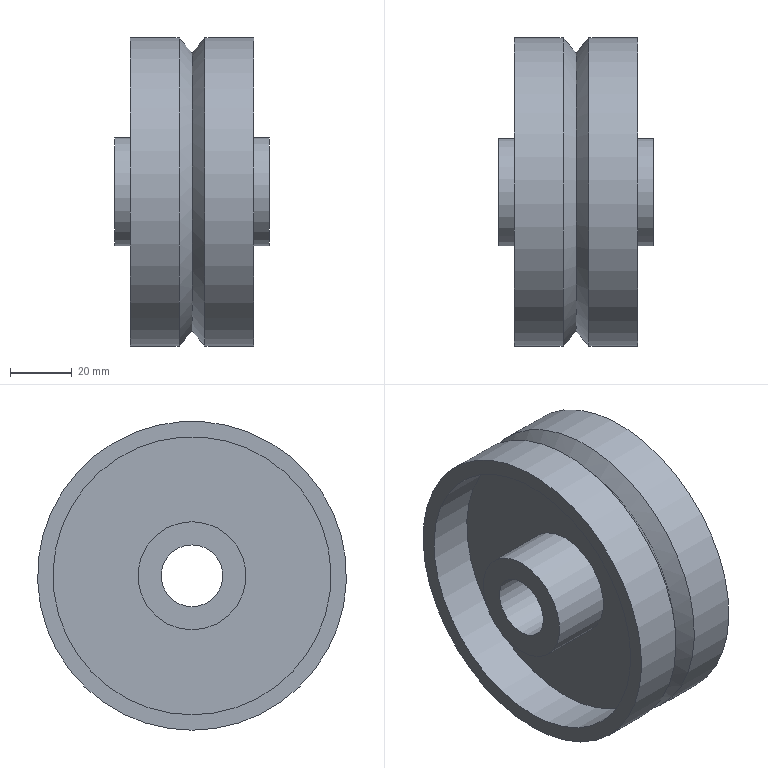Component | NX | RODA_100 | 1 solid | 15 faces | box 50 x 100 x 100 mm | volume 139713 mm3 | cylinder 7 | plane 6 | cone 2 | commonest cylinder face diameters 100 x2 90 x2 35 x2 20 x1
STEP:
#1=CARTESIAN_POINT('',(0.,0.,0.));
#2=DIRECTION('',(0.,0.,1.));
#3=DIRECTION('',(1.,0.,0.));
#4=AXIS2_PLACEMENT_3D('',#1,#2,#3);
#5=CARTESIAN_POINT('',(20.199,0.,-60.));
#6=VERTEX_POINT('',#5);
#7=CARTESIAN_POINT('',(20.199,0.,-10.));
#8=DIRECTION('',(-1.,0.,0.));
#9=DIRECTION('',(0.,0.,-1.));
#10=AXIS2_PLACEMENT_3D('',#7,#8,#9);
#11=CIRCLE('',#10,50.);
#12=CARTESIAN_POINT('',(140.199,0.,-10.));
#13=DIRECTION('',(-1.,0.,0.));
#14=DIRECTION('',(0.,0.,-1.));
#15=AXIS2_PLACEMENT_3D('',#12,#13,#14);
#16=CYLINDRICAL_SURFACE('',#15,50.);
#17=CARTESIAN_POINT('',(0.,120.));
#18=DIRECTION('',(1.,0.));
#19=VECTOR('',#18,1.);
#20=LINE('',#17,#19);
#21=(GEOMETRIC_REPRESENTATION_CONTEXT(2)PARAMETRIC_REPRESENTATION_CONTEXT()REPRESENTATION_CONTEXT('',''));
#22=DEFINITIONAL_REPRESENTATION('',(#20),#21);
#23=PCURVE('',#16,#22);
#24=CARTESIAN_POINT('',(20.199,-50.,-10.));
#25=DIRECTION('',(1.,0.,0.));
#26=DIRECTION('',(0.,0.,1.));
#27=AXIS2_PLACEMENT_3D('',#24,#25,#26);
#28=PLANE('',#27);
#29=CARTESIAN_POINT('',(-50.,-50.));
#30=CARTESIAN_POINT('',(-50.,36.603));
#31=CARTESIAN_POINT('',(25.,-6.699));
#32=CARTESIAN_POINT('',(100.,-50.));
#33=CARTESIAN_POINT('',(25.,-93.301));
#34=CARTESIAN_POINT('',(-50.,-136.603));
#35=CARTESIAN_POINT('',(-50.,-50.));
#36=(BOUNDED_CURVE()B_SPLINE_CURVE(2,(#29,#30,#31,#32,#33,#34,#35),.UNSPECIFIED.,.T.,.F.)B_SPLINE_CURVE_WITH_KNOTS((1,2,2,2,2,1),(-2.094,0.,2.094,4.189,6.283,8.378),.UNSPECIFIED.)CURVE()GEOMETRIC_REPRESENTATION_ITEM()RATIONAL_B_SPLINE_CURVE((1.,0.5,1.,0.5,1.,0.5,1.))REPRESENTATION_ITEM(''));
#37=(GEOMETRIC_REPRESENTATION_CONTEXT(2)PARAMETRIC_REPRESENTATION_CONTEXT()REPRESENTATION_CONTEXT('',''));
#38=DEFINITIONAL_REPRESENTATION('',(#36),#37);
#39=PCURVE('',#28,#38);
#40=SURFACE_CURVE('',#11,(#23,#39),.PCURVE_S1.);
#41=EDGE_CURVE('',#6,#6,#40,.T.);
#42=ORIENTED_EDGE('',*,*,#41,.T.);
#43=CARTESIAN_POINT('',(4.394,0.,-60.));
#44=VERTEX_POINT('',#43);
#45=CARTESIAN_POINT('',(20.199,0.,-60.));
#46=CARTESIAN_POINT('',(4.394,0.,-60.));
#47=B_SPLINE_CURVE_WITH_KNOTS('',1,(#45,#46),.UNSPECIFIED.,.F.,.F.,(2,2),(120.,135.805),.PIECEWISE_BEZIER_KNOTS.);
#48=CARTESIAN_POINT('',(6.283,0.));
#49=DIRECTION('',(0.,1.));
#50=VECTOR('',#49,1.);
#51=LINE('',#48,#50);
#52=(GEOMETRIC_REPRESENTATION_CONTEXT(2)PARAMETRIC_REPRESENTATION_CONTEXT()REPRESENTATION_CONTEXT('',''));
#53=DEFINITIONAL_REPRESENTATION('',(#51),#52);
#54=PCURVE('',#16,#53);
#55=CARTESIAN_POINT('',(0.,0.));
#56=DIRECTION('',(0.,1.));
#57=VECTOR('',#56,1.);
#58=LINE('',#55,#57);
#59=(GEOMETRIC_REPRESENTATION_CONTEXT(2)PARAMETRIC_REPRESENTATION_CONTEXT()REPRESENTATION_CONTEXT('',''));
#60=DEFINITIONAL_REPRESENTATION('',(#58),#59);
#61=PCURVE('',#16,#60);
#62=SEAM_CURVE('',#47,(#54,#61),.PCURVE_S1.);
#63=EDGE_CURVE('',#6,#44,#62,.T.);
#64=ORIENTED_EDGE('',*,*,#63,.T.);
#65=CARTESIAN_POINT('',(4.394,0.,-10.));
#66=DIRECTION('',(-1.,0.,0.));
#67=DIRECTION('',(0.,0.,-1.));
#68=AXIS2_PLACEMENT_3D('',#65,#66,#67);
#69=CIRCLE('',#68,50.);
#70=CARTESIAN_POINT('',(0.,135.805));
#71=DIRECTION('',(1.,0.));
#72=VECTOR('',#71,1.);
#73=LINE('',#70,#72);
#74=(GEOMETRIC_REPRESENTATION_CONTEXT(2)PARAMETRIC_REPRESENTATION_CONTEXT()REPRESENTATION_CONTEXT('',''));
#75=DEFINITIONAL_REPRESENTATION('',(#73),#74);
#76=PCURVE('',#16,#75);
#77=CARTESIAN_POINT('',(0.1986,0.,-10.));
#78=DIRECTION('',(1.,0.,0.));
#79=DIRECTION('',(0.,0.,1.));
#80=AXIS2_PLACEMENT_3D('',#77,#78,#79);
#81=CONICAL_SURFACE('',#80,45.,0.8727);
#82=CARTESIAN_POINT('',(9.425,4.195));
#83=DIRECTION('',(-1.,0.));
#84=VECTOR('',#83,1.);
#85=LINE('',#82,#84);
#86=(GEOMETRIC_REPRESENTATION_CONTEXT(2)PARAMETRIC_REPRESENTATION_CONTEXT()REPRESENTATION_CONTEXT('',''));
#87=DEFINITIONAL_REPRESENTATION('',(#85),#86);
#88=PCURVE('',#81,#87);
#89=SURFACE_CURVE('',#69,(#76,#88),.PCURVE_S1.);
#90=EDGE_CURVE('',#44,#44,#89,.T.);
#91=ORIENTED_EDGE('',*,*,#90,.F.);
#92=ORIENTED_EDGE('',*,*,#63,.F.);
#93=EDGE_LOOP('',(#42,#64,#91,#92));
#94=FACE_BOUND('',#93,.T.);
#95=ADVANCED_FACE('',(#94),#16,.T.);
#96=CARTESIAN_POINT('',(20.199,0.,-55.));
#97=VERTEX_POINT('',#96);
#98=CARTESIAN_POINT('',(20.199,0.,-10.));
#99=DIRECTION('',(-1.,0.,0.));
#100=DIRECTION('',(0.,0.,-1.));
#101=AXIS2_PLACEMENT_3D('',#98,#99,#100);
#102=CIRCLE('',#101,45.);
#103=CARTESIAN_POINT('',(-45.,-50.));
#104=CARTESIAN_POINT('',(-45.,27.942));
#105=CARTESIAN_POINT('',(22.5,-11.029));
#106=CARTESIAN_POINT('',(90.,-50.));
#107=CARTESIAN_POINT('',(22.5,-88.971));
#108=CARTESIAN_POINT('',(-45.,-127.942));
#109=CARTESIAN_POINT('',(-45.,-50.));
#110=(BOUNDED_CURVE()B_SPLINE_CURVE(2,(#103,#104,#105,#106,#107,#108,#109),.UNSPECIFIED.,.T.,.F.)B_SPLINE_CURVE_WITH_KNOTS((1,2,2,2,2,1),(-2.094,0.,2.094,4.189,6.283,8.378),.UNSPECIFIED.)CURVE()GEOMETRIC_REPRESENTATION_ITEM()RATIONAL_B_SPLINE_CURVE((1.,0.5,1.,0.5,1.,0.5,1.))REPRESENTATION_ITEM(''));
#111=(GEOMETRIC_REPRESENTATION_CONTEXT(2)PARAMETRIC_REPRESENTATION_CONTEXT()REPRESENTATION_CONTEXT('',''));
#112=DEFINITIONAL_REPRESENTATION('',(#110),#111);
#113=PCURVE('',#28,#112);
#114=CARTESIAN_POINT('',(140.199,0.,-10.));
#115=DIRECTION('',(-1.,0.,0.));
#116=DIRECTION('',(0.,0.,-1.));
#117=AXIS2_PLACEMENT_3D('',#114,#115,#116);
#118=CYLINDRICAL_SURFACE('',#117,45.);
#119=CARTESIAN_POINT('',(0.,120.));
#120=DIRECTION('',(1.,0.));
#121=VECTOR('',#120,1.);
#122=LINE('',#119,#121);
#123=(GEOMETRIC_REPRESENTATION_CONTEXT(2)PARAMETRIC_REPRESENTATION_CONTEXT()REPRESENTATION_CONTEXT('',''));
#124=DEFINITIONAL_REPRESENTATION('',(#122),#123);
#125=PCURVE('',#118,#124);
#126=SURFACE_CURVE('',#102,(#113,#125),.PCURVE_S1.);
#127=EDGE_CURVE('',#97,#97,#126,.T.);
#128=ORIENTED_EDGE('',*,*,#127,.T.);
#129=EDGE_LOOP('',(#128));
#130=FACE_BOUND('',#129,.T.);
#131=ORIENTED_EDGE('',*,*,#41,.F.);
#132=EDGE_LOOP('',(#131));
#133=FACE_BOUND('',#132,.T.);
#134=ADVANCED_FACE('',(#130,#133),#28,.T.);
#135=CARTESIAN_POINT('',(5.199,0.,-55.));
#136=VERTEX_POINT('',#135);
#137=CARTESIAN_POINT('',(5.199,0.,-10.));
#138=DIRECTION('',(-1.,0.,0.));
#139=DIRECTION('',(0.,0.,-1.));
#140=AXIS2_PLACEMENT_3D('',#137,#138,#139);
#141=CIRCLE('',#140,45.);
#142=CARTESIAN_POINT('',(0.,135.));
#143=DIRECTION('',(1.,0.));
#144=VECTOR('',#143,1.);
#145=LINE('',#142,#144);
#146=(GEOMETRIC_REPRESENTATION_CONTEXT(2)PARAMETRIC_REPRESENTATION_CONTEXT()REPRESENTATION_CONTEXT('',''));
#147=DEFINITIONAL_REPRESENTATION('',(#145),#146);
#148=PCURVE('',#118,#147);
#149=CARTESIAN_POINT('',(5.199,-45.,-10.));
#150=DIRECTION('',(1.,0.,0.));
#151=DIRECTION('',(0.,0.,1.));
#152=AXIS2_PLACEMENT_3D('',#149,#150,#151);
#153=PLANE('',#152);
#154=CARTESIAN_POINT('',(-45.,-45.));
#155=CARTESIAN_POINT('',(-45.,32.942));
#156=CARTESIAN_POINT('',(22.5,-6.029));
#157=CARTESIAN_POINT('',(90.,-45.));
#158=CARTESIAN_POINT('',(22.5,-83.971));
#159=CARTESIAN_POINT('',(-45.,-122.942));
#160=CARTESIAN_POINT('',(-45.,-45.));
#161=(BOUNDED_CURVE()B_SPLINE_CURVE(2,(#154,#155,#156,#157,#158,#159,#160),.UNSPECIFIED.,.T.,.F.)B_SPLINE_CURVE_WITH_KNOTS((1,2,2,2,2,1),(-2.094,0.,2.094,4.189,6.283,8.378),.UNSPECIFIED.)CURVE()GEOMETRIC_REPRESENTATION_ITEM()RATIONAL_B_SPLINE_CURVE((1.,0.5,1.,0.5,1.,0.5,1.))REPRESENTATION_ITEM(''));
#162=(GEOMETRIC_REPRESENTATION_CONTEXT(2)PARAMETRIC_REPRESENTATION_CONTEXT()REPRESENTATION_CONTEXT('',''));
#163=DEFINITIONAL_REPRESENTATION('',(#161),#162);
#164=PCURVE('',#153,#163);
#165=SURFACE_CURVE('',#141,(#148,#164),.PCURVE_S1.);
#166=EDGE_CURVE('',#136,#136,#165,.T.);
#167=ORIENTED_EDGE('',*,*,#166,.F.);
#168=CARTESIAN_POINT('',(20.199,0.,-55.));
#169=CARTESIAN_POINT('',(5.199,0.,-55.));
#170=B_SPLINE_CURVE_WITH_KNOTS('',1,(#168,#169),.UNSPECIFIED.,.F.,.F.,(2,2),(120.,135.),.PIECEWISE_BEZIER_KNOTS.);
#171=CARTESIAN_POINT('',(0.,0.));
#172=DIRECTION('',(0.,1.));
#173=VECTOR('',#172,1.);
#174=LINE('',#171,#173);
#175=(GEOMETRIC_REPRESENTATION_CONTEXT(2)PARAMETRIC_REPRESENTATION_CONTEXT()REPRESENTATION_CONTEXT('',''));
#176=DEFINITIONAL_REPRESENTATION('',(#174),#175);
#177=PCURVE('',#118,#176);
#178=CARTESIAN_POINT('',(6.283,0.));
#179=DIRECTION('',(0.,1.));
#180=VECTOR('',#179,1.);
#181=LINE('',#178,#180);
#182=(GEOMETRIC_REPRESENTATION_CONTEXT(2)PARAMETRIC_REPRESENTATION_CONTEXT()REPRESENTATION_CONTEXT('',''));
#183=DEFINITIONAL_REPRESENTATION('',(#181),#182);
#184=PCURVE('',#118,#183);
#185=SEAM_CURVE('',#170,(#177,#184),.PCURVE_S1.);
#186=EDGE_CURVE('',#97,#136,#185,.T.);
#187=ORIENTED_EDGE('',*,*,#186,.F.);
#188=ORIENTED_EDGE('',*,*,#127,.T.);
#189=ORIENTED_EDGE('',*,*,#186,.T.);
#190=EDGE_LOOP('',(#167,#187,#188,#189));
#191=FACE_BOUND('',#190,.F.);
#192=ADVANCED_FACE('',(#191),#118,.F.);
#193=CARTESIAN_POINT('',(5.199,0.,-27.5));
#194=VERTEX_POINT('',#193);
#195=CARTESIAN_POINT('',(5.199,0.,-10.));
#196=DIRECTION('',(-1.,0.,0.));
#197=DIRECTION('',(0.,0.,-1.));
#198=AXIS2_PLACEMENT_3D('',#195,#196,#197);
#199=CIRCLE('',#198,17.5);
#200=CARTESIAN_POINT('',(-17.5,-45.));
#201=CARTESIAN_POINT('',(-17.5,-14.689));
#202=CARTESIAN_POINT('',(8.75,-29.845));
#203=CARTESIAN_POINT('',(35.,-45.));
#204=CARTESIAN_POINT('',(8.75,-60.155));
#205=CARTESIAN_POINT('',(-17.5,-75.311));
#206=CARTESIAN_POINT('',(-17.5,-45.));
#207=(BOUNDED_CURVE()B_SPLINE_CURVE(2,(#200,#201,#202,#203,#204,#205,#206),.UNSPECIFIED.,.T.,.F.)B_SPLINE_CURVE_WITH_KNOTS((1,2,2,2,2,1),(-2.094,0.,2.094,4.189,6.283,8.378),.UNSPECIFIED.)CURVE()GEOMETRIC_REPRESENTATION_ITEM()RATIONAL_B_SPLINE_CURVE((1.,0.5,1.,0.5,1.,0.5,1.))REPRESENTATION_ITEM(''));
#208=(GEOMETRIC_REPRESENTATION_CONTEXT(2)PARAMETRIC_REPRESENTATION_CONTEXT()REPRESENTATION_CONTEXT('',''));
#209=DEFINITIONAL_REPRESENTATION('',(#207),#208);
#210=PCURVE('',#153,#209);
#211=CARTESIAN_POINT('',(140.199,0.,-10.));
#212=DIRECTION('',(-1.,0.,0.));
#213=DIRECTION('',(0.,0.,-1.));
#214=AXIS2_PLACEMENT_3D('',#211,#212,#213);
#215=CYLINDRICAL_SURFACE('',#214,17.5);
#216=CARTESIAN_POINT('',(0.,135.));
#217=DIRECTION('',(1.,0.));
#218=VECTOR('',#217,1.);
#219=LINE('',#216,#218);
#220=(GEOMETRIC_REPRESENTATION_CONTEXT(2)PARAMETRIC_REPRESENTATION_CONTEXT()REPRESENTATION_CONTEXT('',''));
#221=DEFINITIONAL_REPRESENTATION('',(#219),#220);
#222=PCURVE('',#215,#221);
#223=SURFACE_CURVE('',#199,(#210,#222),.PCURVE_S1.);
#224=EDGE_CURVE('',#194,#194,#223,.T.);
#225=ORIENTED_EDGE('',*,*,#224,.T.);
#226=EDGE_LOOP('',(#225));
#227=FACE_BOUND('',#226,.T.);
#228=ORIENTED_EDGE('',*,*,#166,.F.);
#229=EDGE_LOOP('',(#228));
#230=FACE_BOUND('',#229,.T.);
#231=ADVANCED_FACE('',(#227,#230),#153,.T.);
#232=CARTESIAN_POINT('',(25.199,0.,-27.5));
#233=VERTEX_POINT('',#232);
#234=CARTESIAN_POINT('',(25.199,0.,-10.));
#235=DIRECTION('',(-1.,0.,0.));
#236=DIRECTION('',(0.,0.,-1.));
#237=AXIS2_PLACEMENT_3D('',#234,#235,#236);
#238=CIRCLE('',#237,17.5);
#239=CARTESIAN_POINT('',(0.,115.));
#240=DIRECTION('',(1.,0.));
#241=VECTOR('',#240,1.);
#242=LINE('',#239,#241);
#243=(GEOMETRIC_REPRESENTATION_CONTEXT(2)PARAMETRIC_REPRESENTATION_CONTEXT()REPRESENTATION_CONTEXT('',''));
#244=DEFINITIONAL_REPRESENTATION('',(#242),#243);
#245=PCURVE('',#215,#244);
#246=CARTESIAN_POINT('',(25.199,-17.5,-10.));
#247=DIRECTION('',(1.,0.,0.));
#248=DIRECTION('',(0.,0.,1.));
#249=AXIS2_PLACEMENT_3D('',#246,#247,#248);
#250=PLANE('',#249);
#251=CARTESIAN_POINT('',(-17.5,-17.5));
#252=CARTESIAN_POINT('',(-17.5,12.811));
#253=CARTESIAN_POINT('',(8.75,-2.345));
#254=CARTESIAN_POINT('',(35.,-17.5));
#255=CARTESIAN_POINT('',(8.75,-32.655));
#256=CARTESIAN_POINT('',(-17.5,-47.811));
#257=CARTESIAN_POINT('',(-17.5,-17.5));
#258=(BOUNDED_CURVE()B_SPLINE_CURVE(2,(#251,#252,#253,#254,#255,#256,#257),.UNSPECIFIED.,.T.,.F.)B_SPLINE_CURVE_WITH_KNOTS((1,2,2,2,2,1),(-2.094,0.,2.094,4.189,6.283,8.378),.UNSPECIFIED.)CURVE()GEOMETRIC_REPRESENTATION_ITEM()RATIONAL_B_SPLINE_CURVE((1.,0.5,1.,0.5,1.,0.5,1.))REPRESENTATION_ITEM(''));
#259=(GEOMETRIC_REPRESENTATION_CONTEXT(2)PARAMETRIC_REPRESENTATION_CONTEXT()REPRESENTATION_CONTEXT('',''));
#260=DEFINITIONAL_REPRESENTATION('',(#258),#259);
#261=PCURVE('',#250,#260);
#262=SURFACE_CURVE('',#238,(#245,#261),.PCURVE_S1.);
#263=EDGE_CURVE('',#233,#233,#262,.T.);
#264=ORIENTED_EDGE('',*,*,#263,.T.);
#265=CARTESIAN_POINT('',(25.199,0.,-27.5));
#266=CARTESIAN_POINT('',(5.199,0.,-27.5));
#267=B_SPLINE_CURVE_WITH_KNOTS('',1,(#265,#266),.UNSPECIFIED.,.F.,.F.,(2,2),(115.,135.),.PIECEWISE_BEZIER_KNOTS.);
#268=CARTESIAN_POINT('',(6.283,0.));
#269=DIRECTION('',(0.,1.));
#270=VECTOR('',#269,1.);
#271=LINE('',#268,#270);
#272=(GEOMETRIC_REPRESENTATION_CONTEXT(2)PARAMETRIC_REPRESENTATION_CONTEXT()REPRESENTATION_CONTEXT('',''));
#273=DEFINITIONAL_REPRESENTATION('',(#271),#272);
#274=PCURVE('',#215,#273);
#275=CARTESIAN_POINT('',(0.,0.));
#276=DIRECTION('',(0.,1.));
#277=VECTOR('',#276,1.);
#278=LINE('',#275,#277);
#279=(GEOMETRIC_REPRESENTATION_CONTEXT(2)PARAMETRIC_REPRESENTATION_CONTEXT()REPRESENTATION_CONTEXT('',''));
#280=DEFINITIONAL_REPRESENTATION('',(#278),#279);
#281=PCURVE('',#215,#280);
#282=SEAM_CURVE('',#267,(#274,#281),.PCURVE_S1.);
#283=EDGE_CURVE('',#233,#194,#282,.T.);
#284=ORIENTED_EDGE('',*,*,#283,.T.);
#285=ORIENTED_EDGE('',*,*,#224,.F.);
#286=ORIENTED_EDGE('',*,*,#283,.F.);
#287=EDGE_LOOP('',(#264,#284,#285,#286));
#288=FACE_BOUND('',#287,.T.);
#289=ADVANCED_FACE('',(#288),#215,.T.);
#290=CARTESIAN_POINT('',(25.199,0.,-20.));
#291=VERTEX_POINT('',#290);
#292=CARTESIAN_POINT('',(25.199,0.,-10.));
#293=DIRECTION('',(-1.,0.,0.));
#294=DIRECTION('',(0.,0.,-1.));
#295=AXIS2_PLACEMENT_3D('',#292,#293,#294);
#296=CIRCLE('',#295,10.);
#297=CARTESIAN_POINT('',(-10.,-17.5));
#298=CARTESIAN_POINT('',(-10.,-0.1795));
#299=CARTESIAN_POINT('',(5.,-8.84));
#300=CARTESIAN_POINT('',(20.,-17.5));
#301=CARTESIAN_POINT('',(5.,-26.16));
#302=CARTESIAN_POINT('',(-10.,-34.821));
#303=CARTESIAN_POINT('',(-10.,-17.5));
#304=(BOUNDED_CURVE()B_SPLINE_CURVE(2,(#297,#298,#299,#300,#301,#302,#303),.UNSPECIFIED.,.T.,.F.)B_SPLINE_CURVE_WITH_KNOTS((1,2,2,2,2,1),(-2.094,0.,2.094,4.189,6.283,8.378),.UNSPECIFIED.)CURVE()GEOMETRIC_REPRESENTATION_ITEM()RATIONAL_B_SPLINE_CURVE((1.,0.5,1.,0.5,1.,0.5,1.))REPRESENTATION_ITEM(''));
#305=(GEOMETRIC_REPRESENTATION_CONTEXT(2)PARAMETRIC_REPRESENTATION_CONTEXT()REPRESENTATION_CONTEXT('',''));
#306=DEFINITIONAL_REPRESENTATION('',(#304),#305);
#307=PCURVE('',#250,#306);
#308=CARTESIAN_POINT('',(140.199,0.,-10.));
#309=DIRECTION('',(-1.,0.,0.));
#310=DIRECTION('',(0.,0.,-1.));
#311=AXIS2_PLACEMENT_3D('',#308,#309,#310);
#312=CYLINDRICAL_SURFACE('',#311,10.);
#313=CARTESIAN_POINT('',(0.,115.));
#314=DIRECTION('',(1.,0.));
#315=VECTOR('',#314,1.);
#316=LINE('',#313,#315);
#317=(GEOMETRIC_REPRESENTATION_CONTEXT(2)PARAMETRIC_REPRESENTATION_CONTEXT()REPRESENTATION_CONTEXT('',''));
#318=DEFINITIONAL_REPRESENTATION('',(#316),#317);
#319=PCURVE('',#312,#318);
#320=SURFACE_CURVE('',#296,(#307,#319),.PCURVE_S1.);
#321=EDGE_CURVE('',#291,#291,#320,.T.);
#322=ORIENTED_EDGE('',*,*,#321,.T.);
#323=EDGE_LOOP('',(#322));
#324=FACE_BOUND('',#323,.T.);
#325=ORIENTED_EDGE('',*,*,#263,.F.);
#326=EDGE_LOOP('',(#325));
#327=FACE_BOUND('',#326,.T.);
#328=ADVANCED_FACE('',(#324,#327),#250,.T.);
#329=CARTESIAN_POINT('',(-24.801,0.,-20.));
#330=VERTEX_POINT('',#329);
#331=CARTESIAN_POINT('',(-24.801,0.,-10.));
#332=DIRECTION('',(-1.,0.,0.));
#333=DIRECTION('',(0.,0.,-1.));
#334=AXIS2_PLACEMENT_3D('',#331,#332,#333);
#335=CIRCLE('',#334,10.);
#336=CARTESIAN_POINT('',(0.,165.));
#337=DIRECTION('',(1.,0.));
#338=VECTOR('',#337,1.);
#339=LINE('',#336,#338);
#340=(GEOMETRIC_REPRESENTATION_CONTEXT(2)PARAMETRIC_REPRESENTATION_CONTEXT()REPRESENTATION_CONTEXT('',''));
#341=DEFINITIONAL_REPRESENTATION('',(#339),#340);
#342=PCURVE('',#312,#341);
#343=CARTESIAN_POINT('',(-24.801,-10.,-10.));
#344=DIRECTION('',(-1.,0.,0.));
#345=DIRECTION('',(0.,0.,-1.));
#346=AXIS2_PLACEMENT_3D('',#343,#344,#345);
#347=PLANE('',#346);
#348=CARTESIAN_POINT('',(0.,-10.));
#349=DIRECTION('',(1.,0.));
#350=AXIS2_PLACEMENT_2D('',#348,#349);
#351=CIRCLE('',#350,10.);
#352=(GEOMETRIC_REPRESENTATION_CONTEXT(2)PARAMETRIC_REPRESENTATION_CONTEXT()REPRESENTATION_CONTEXT('',''));
#353=DEFINITIONAL_REPRESENTATION('',(#351),#352);
#354=PCURVE('',#347,#353);
#355=SURFACE_CURVE('',#335,(#342,#354),.PCURVE_S1.);
#356=EDGE_CURVE('',#330,#330,#355,.T.);
#357=ORIENTED_EDGE('',*,*,#356,.F.);
#358=CARTESIAN_POINT('',(25.199,0.,-20.));
#359=CARTESIAN_POINT('',(-24.801,0.,-20.));
#360=B_SPLINE_CURVE_WITH_KNOTS('',1,(#358,#359),.UNSPECIFIED.,.F.,.F.,(2,2),(115.,165.),.PIECEWISE_BEZIER_KNOTS.);
#361=CARTESIAN_POINT('',(0.,0.));
#362=DIRECTION('',(0.,1.));
#363=VECTOR('',#362,1.);
#364=LINE('',#361,#363);
#365=(GEOMETRIC_REPRESENTATION_CONTEXT(2)PARAMETRIC_REPRESENTATION_CONTEXT()REPRESENTATION_CONTEXT('',''));
#366=DEFINITIONAL_REPRESENTATION('',(#364),#365);
#367=PCURVE('',#312,#366);
#368=CARTESIAN_POINT('',(6.283,0.));
#369=DIRECTION('',(0.,1.));
#370=VECTOR('',#369,1.);
#371=LINE('',#368,#370);
#372=(GEOMETRIC_REPRESENTATION_CONTEXT(2)PARAMETRIC_REPRESENTATION_CONTEXT()REPRESENTATION_CONTEXT('',''));
#373=DEFINITIONAL_REPRESENTATION('',(#371),#372);
#374=PCURVE('',#312,#373);
#375=SEAM_CURVE('',#360,(#367,#374),.PCURVE_S1.);
#376=EDGE_CURVE('',#291,#330,#375,.T.);
#377=ORIENTED_EDGE('',*,*,#376,.F.);
#378=ORIENTED_EDGE('',*,*,#321,.T.);
#379=ORIENTED_EDGE('',*,*,#376,.T.);
#380=EDGE_LOOP('',(#357,#377,#378,#379));
#381=FACE_BOUND('',#380,.F.);
#382=ADVANCED_FACE('',(#381),#312,.F.);
#383=CARTESIAN_POINT('',(-24.801,0.,-27.5));
#384=VERTEX_POINT('',#383);
#385=CARTESIAN_POINT('',(-24.801,0.,-10.));
#386=DIRECTION('',(-1.,0.,0.));
#387=DIRECTION('',(0.,0.,-1.));
#388=AXIS2_PLACEMENT_3D('',#385,#386,#387);
#389=CIRCLE('',#388,17.5);
#390=CARTESIAN_POINT('',(0.,-10.));
#391=DIRECTION('',(1.,0.));
#392=AXIS2_PLACEMENT_2D('',#390,#391);
#393=CIRCLE('',#392,17.5);
#394=(GEOMETRIC_REPRESENTATION_CONTEXT(2)PARAMETRIC_REPRESENTATION_CONTEXT()REPRESENTATION_CONTEXT('',''));
#395=DEFINITIONAL_REPRESENTATION('',(#393),#394);
#396=PCURVE('',#347,#395);
#397=CARTESIAN_POINT('',(140.199,0.,-10.));
#398=DIRECTION('',(-1.,0.,0.));
#399=DIRECTION('',(0.,0.,-1.));
#400=AXIS2_PLACEMENT_3D('',#397,#398,#399);
#401=CYLINDRICAL_SURFACE('',#400,17.5);
#402=CARTESIAN_POINT('',(0.,165.));
#403=DIRECTION('',(1.,0.));
#404=VECTOR('',#403,1.);
#405=LINE('',#402,#404);
#406=(GEOMETRIC_REPRESENTATION_CONTEXT(2)PARAMETRIC_REPRESENTATION_CONTEXT()REPRESENTATION_CONTEXT('',''));
#407=DEFINITIONAL_REPRESENTATION('',(#405),#406);
#408=PCURVE('',#401,#407);
#409=SURFACE_CURVE('',#389,(#396,#408),.PCURVE_S1.);
#410=EDGE_CURVE('',#384,#384,#409,.T.);
#411=ORIENTED_EDGE('',*,*,#410,.T.);
#412=EDGE_LOOP('',(#411));
#413=FACE_BOUND('',#412,.T.);
#414=ORIENTED_EDGE('',*,*,#356,.F.);
#415=EDGE_LOOP('',(#414));
#416=FACE_BOUND('',#415,.T.);
#417=ADVANCED_FACE('',(#413,#416),#347,.T.);
#418=CARTESIAN_POINT('',(-4.801,0.,-27.5));
#419=VERTEX_POINT('',#418);
#420=CARTESIAN_POINT('',(-4.801,0.,-10.));
#421=DIRECTION('',(-1.,0.,0.));
#422=DIRECTION('',(0.,0.,-1.));
#423=AXIS2_PLACEMENT_3D('',#420,#421,#422);
#424=CIRCLE('',#423,17.5);
#425=CARTESIAN_POINT('',(0.,145.));
#426=DIRECTION('',(1.,0.));
#427=VECTOR('',#426,1.);
#428=LINE('',#425,#427);
#429=(GEOMETRIC_REPRESENTATION_CONTEXT(2)PARAMETRIC_REPRESENTATION_CONTEXT()REPRESENTATION_CONTEXT('',''));
#430=DEFINITIONAL_REPRESENTATION('',(#428),#429);
#431=PCURVE('',#401,#430);
#432=CARTESIAN_POINT('',(-4.801,-17.5,-10.));
#433=DIRECTION('',(-1.,0.,0.));
#434=DIRECTION('',(0.,0.,-1.));
#435=AXIS2_PLACEMENT_3D('',#432,#433,#434);
#436=PLANE('',#435);
#437=CARTESIAN_POINT('',(0.,-17.5));
#438=DIRECTION('',(1.,0.));
#439=AXIS2_PLACEMENT_2D('',#437,#438);
#440=CIRCLE('',#439,17.5);
#441=(GEOMETRIC_REPRESENTATION_CONTEXT(2)PARAMETRIC_REPRESENTATION_CONTEXT()REPRESENTATION_CONTEXT('',''));
#442=DEFINITIONAL_REPRESENTATION('',(#440),#441);
#443=PCURVE('',#436,#442);
#444=SURFACE_CURVE('',#424,(#431,#443),.PCURVE_S1.);
#445=EDGE_CURVE('',#419,#419,#444,.T.);
#446=ORIENTED_EDGE('',*,*,#445,.T.);
#447=CARTESIAN_POINT('',(-4.801,0.,-27.5));
#448=CARTESIAN_POINT('',(-24.801,0.,-27.5));
#449=B_SPLINE_CURVE_WITH_KNOTS('',1,(#447,#448),.UNSPECIFIED.,.F.,.F.,(2,2),(145.,165.),.PIECEWISE_BEZIER_KNOTS.);
#450=CARTESIAN_POINT('',(6.283,0.));
#451=DIRECTION('',(0.,1.));
#452=VECTOR('',#451,1.);
#453=LINE('',#450,#452);
#454=(GEOMETRIC_REPRESENTATION_CONTEXT(2)PARAMETRIC_REPRESENTATION_CONTEXT()REPRESENTATION_CONTEXT('',''));
#455=DEFINITIONAL_REPRESENTATION('',(#453),#454);
#456=PCURVE('',#401,#455);
#457=CARTESIAN_POINT('',(0.,0.));
#458=DIRECTION('',(0.,1.));
#459=VECTOR('',#458,1.);
#460=LINE('',#457,#459);
#461=(GEOMETRIC_REPRESENTATION_CONTEXT(2)PARAMETRIC_REPRESENTATION_CONTEXT()REPRESENTATION_CONTEXT('',''));
#462=DEFINITIONAL_REPRESENTATION('',(#460),#461);
#463=PCURVE('',#401,#462);
#464=SEAM_CURVE('',#449,(#456,#463),.PCURVE_S1.);
#465=EDGE_CURVE('',#419,#384,#464,.T.);
#466=ORIENTED_EDGE('',*,*,#465,.T.);
#467=ORIENTED_EDGE('',*,*,#410,.F.);
#468=ORIENTED_EDGE('',*,*,#465,.F.);
#469=EDGE_LOOP('',(#446,#466,#467,#468));
#470=FACE_BOUND('',#469,.T.);
#471=ADVANCED_FACE('',(#470),#401,.T.);
#472=CARTESIAN_POINT('',(-4.801,0.,-55.));
#473=VERTEX_POINT('',#472);
#474=CARTESIAN_POINT('',(-4.801,0.,-10.));
#475=DIRECTION('',(-1.,0.,0.));
#476=DIRECTION('',(0.,0.,-1.));
#477=AXIS2_PLACEMENT_3D('',#474,#475,#476);
#478=CIRCLE('',#477,45.);
#479=CARTESIAN_POINT('',(0.,-17.5));
#480=DIRECTION('',(1.,0.));
#481=AXIS2_PLACEMENT_2D('',#479,#480);
#482=CIRCLE('',#481,45.);
#483=(GEOMETRIC_REPRESENTATION_CONTEXT(2)PARAMETRIC_REPRESENTATION_CONTEXT()REPRESENTATION_CONTEXT('',''));
#484=DEFINITIONAL_REPRESENTATION('',(#482),#483);
#485=PCURVE('',#436,#484);
#486=CARTESIAN_POINT('',(140.199,0.,-10.));
#487=DIRECTION('',(-1.,0.,0.));
#488=DIRECTION('',(0.,0.,-1.));
#489=AXIS2_PLACEMENT_3D('',#486,#487,#488);
#490=CYLINDRICAL_SURFACE('',#489,45.);
#491=CARTESIAN_POINT('',(0.,145.));
#492=DIRECTION('',(1.,0.));
#493=VECTOR('',#492,1.);
#494=LINE('',#491,#493);
#495=(GEOMETRIC_REPRESENTATION_CONTEXT(2)PARAMETRIC_REPRESENTATION_CONTEXT()REPRESENTATION_CONTEXT('',''));
#496=DEFINITIONAL_REPRESENTATION('',(#494),#495);
#497=PCURVE('',#490,#496);
#498=SURFACE_CURVE('',#478,(#485,#497),.PCURVE_S1.);
#499=EDGE_CURVE('',#473,#473,#498,.T.);
#500=ORIENTED_EDGE('',*,*,#499,.T.);
#501=EDGE_LOOP('',(#500));
#502=FACE_BOUND('',#501,.T.);
#503=ORIENTED_EDGE('',*,*,#445,.F.);
#504=EDGE_LOOP('',(#503));
#505=FACE_BOUND('',#504,.T.);
#506=ADVANCED_FACE('',(#502,#505),#436,.T.);
#507=CARTESIAN_POINT('',(-19.801,0.,-55.));
#508=VERTEX_POINT('',#507);
#509=CARTESIAN_POINT('',(-19.801,0.,-10.));
#510=DIRECTION('',(-1.,0.,0.));
#511=DIRECTION('',(0.,0.,-1.));
#512=AXIS2_PLACEMENT_3D('',#509,#510,#511);
#513=CIRCLE('',#512,45.);
#514=CARTESIAN_POINT('',(0.,160.));
#515=DIRECTION('',(1.,0.));
#516=VECTOR('',#515,1.);
#517=LINE('',#514,#516);
#518=(GEOMETRIC_REPRESENTATION_CONTEXT(2)PARAMETRIC_REPRESENTATION_CONTEXT()REPRESENTATION_CONTEXT('',''));
#519=DEFINITIONAL_REPRESENTATION('',(#517),#518);
#520=PCURVE('',#490,#519);
#521=CARTESIAN_POINT('',(-19.801,-45.,-10.));
#522=DIRECTION('',(-1.,0.,0.));
#523=DIRECTION('',(0.,0.,-1.));
#524=AXIS2_PLACEMENT_3D('',#521,#522,#523);
#525=PLANE('',#524);
#526=CARTESIAN_POINT('',(0.,-45.));
#527=DIRECTION('',(1.,0.));
#528=AXIS2_PLACEMENT_2D('',#526,#527);
#529=CIRCLE('',#528,45.);
#530=(GEOMETRIC_REPRESENTATION_CONTEXT(2)PARAMETRIC_REPRESENTATION_CONTEXT()REPRESENTATION_CONTEXT('',''));
#531=DEFINITIONAL_REPRESENTATION('',(#529),#530);
#532=PCURVE('',#525,#531);
#533=SURFACE_CURVE('',#513,(#520,#532),.PCURVE_S1.);
#534=EDGE_CURVE('',#508,#508,#533,.T.);
#535=ORIENTED_EDGE('',*,*,#534,.F.);
#536=CARTESIAN_POINT('',(-4.801,0.,-55.));
#537=CARTESIAN_POINT('',(-19.801,0.,-55.));
#538=B_SPLINE_CURVE_WITH_KNOTS('',1,(#536,#537),.UNSPECIFIED.,.F.,.F.,(2,2),(145.,160.),.PIECEWISE_BEZIER_KNOTS.);
#539=CARTESIAN_POINT('',(0.,0.));
#540=DIRECTION('',(0.,1.));
#541=VECTOR('',#540,1.);
#542=LINE('',#539,#541);
#543=(GEOMETRIC_REPRESENTATION_CONTEXT(2)PARAMETRIC_REPRESENTATION_CONTEXT()REPRESENTATION_CONTEXT('',''));
#544=DEFINITIONAL_REPRESENTATION('',(#542),#543);
#545=PCURVE('',#490,#544);
#546=CARTESIAN_POINT('',(6.283,0.));
#547=DIRECTION('',(0.,1.));
#548=VECTOR('',#547,1.);
#549=LINE('',#546,#548);
#550=(GEOMETRIC_REPRESENTATION_CONTEXT(2)PARAMETRIC_REPRESENTATION_CONTEXT()REPRESENTATION_CONTEXT('',''));
#551=DEFINITIONAL_REPRESENTATION('',(#549),#550);
#552=PCURVE('',#490,#551);
#553=SEAM_CURVE('',#538,(#545,#552),.PCURVE_S1.);
#554=EDGE_CURVE('',#473,#508,#553,.T.);
#555=ORIENTED_EDGE('',*,*,#554,.F.);
#556=ORIENTED_EDGE('',*,*,#499,.T.);
#557=ORIENTED_EDGE('',*,*,#554,.T.);
#558=EDGE_LOOP('',(#535,#555,#556,#557));
#559=FACE_BOUND('',#558,.F.);
#560=ADVANCED_FACE('',(#559),#490,.F.);
#561=CARTESIAN_POINT('',(-19.801,0.,-60.));
#562=VERTEX_POINT('',#561);
#563=CARTESIAN_POINT('',(-19.801,0.,-10.));
#564=DIRECTION('',(-1.,0.,0.));
#565=DIRECTION('',(0.,0.,-1.));
#566=AXIS2_PLACEMENT_3D('',#563,#564,#565);
#567=CIRCLE('',#566,50.);
#568=CARTESIAN_POINT('',(0.,-45.));
#569=DIRECTION('',(1.,0.));
#570=AXIS2_PLACEMENT_2D('',#568,#569);
#571=CIRCLE('',#570,50.);
#572=(GEOMETRIC_REPRESENTATION_CONTEXT(2)PARAMETRIC_REPRESENTATION_CONTEXT()REPRESENTATION_CONTEXT('',''));
#573=DEFINITIONAL_REPRESENTATION('',(#571),#572);
#574=PCURVE('',#525,#573);
#575=CARTESIAN_POINT('',(140.199,0.,-10.));
#576=DIRECTION('',(-1.,0.,0.));
#577=DIRECTION('',(0.,0.,-1.));
#578=AXIS2_PLACEMENT_3D('',#575,#576,#577);
#579=CYLINDRICAL_SURFACE('',#578,50.);
#580=CARTESIAN_POINT('',(0.,160.));
#581=DIRECTION('',(1.,0.));
#582=VECTOR('',#581,1.);
#583=LINE('',#580,#582);
#584=(GEOMETRIC_REPRESENTATION_CONTEXT(2)PARAMETRIC_REPRESENTATION_CONTEXT()REPRESENTATION_CONTEXT('',''));
#585=DEFINITIONAL_REPRESENTATION('',(#583),#584);
#586=PCURVE('',#579,#585);
#587=SURFACE_CURVE('',#567,(#574,#586),.PCURVE_S1.);
#588=EDGE_CURVE('',#562,#562,#587,.T.);
#589=ORIENTED_EDGE('',*,*,#588,.T.);
#590=EDGE_LOOP('',(#589));
#591=FACE_BOUND('',#590,.T.);
#592=ORIENTED_EDGE('',*,*,#534,.F.);
#593=EDGE_LOOP('',(#592));
#594=FACE_BOUND('',#593,.T.);
#595=ADVANCED_FACE('',(#591,#594),#525,.T.);
#596=CARTESIAN_POINT('',(-3.997,0.,-60.));
#597=VERTEX_POINT('',#596);
#598=CARTESIAN_POINT('',(-3.997,0.,-10.));
#599=DIRECTION('',(-1.,0.,0.));
#600=DIRECTION('',(0.,0.,-1.));
#601=AXIS2_PLACEMENT_3D('',#598,#599,#600);
#602=CIRCLE('',#601,50.);
#603=CARTESIAN_POINT('',(0.,144.195));
#604=DIRECTION('',(1.,0.));
#605=VECTOR('',#604,1.);
#606=LINE('',#603,#605);
#607=(GEOMETRIC_REPRESENTATION_CONTEXT(2)PARAMETRIC_REPRESENTATION_CONTEXT()REPRESENTATION_CONTEXT('',''));
#608=DEFINITIONAL_REPRESENTATION('',(#606),#607);
#609=PCURVE('',#579,#608);
#610=CARTESIAN_POINT('',(-3.997,0.,-10.));
#611=DIRECTION('',(-1.,0.,0.));
#612=DIRECTION('',(0.,0.,-1.));
#613=AXIS2_PLACEMENT_3D('',#610,#611,#612);
#614=CONICAL_SURFACE('',#613,50.,0.8727);
#615=CARTESIAN_POINT('',(0.,0.));
#616=DIRECTION('',(1.,0.));
#617=VECTOR('',#616,1.);
#618=LINE('',#615,#617);
#619=(GEOMETRIC_REPRESENTATION_CONTEXT(2)PARAMETRIC_REPRESENTATION_CONTEXT()REPRESENTATION_CONTEXT('',''));
#620=DEFINITIONAL_REPRESENTATION('',(#618),#619);
#621=PCURVE('',#614,#620);
#622=SURFACE_CURVE('',#602,(#609,#621),.PCURVE_S1.);
#623=EDGE_CURVE('',#597,#597,#622,.T.);
#624=ORIENTED_EDGE('',*,*,#623,.T.);
#625=CARTESIAN_POINT('',(-3.997,0.,-60.));
#626=CARTESIAN_POINT('',(-19.801,0.,-60.));
#627=B_SPLINE_CURVE_WITH_KNOTS('',1,(#625,#626),.UNSPECIFIED.,.F.,.F.,(2,2),(144.195,160.),.PIECEWISE_BEZIER_KNOTS.);
#628=CARTESIAN_POINT('',(6.283,0.));
#629=DIRECTION('',(0.,1.));
#630=VECTOR('',#629,1.);
#631=LINE('',#628,#630);
#632=(GEOMETRIC_REPRESENTATION_CONTEXT(2)PARAMETRIC_REPRESENTATION_CONTEXT()REPRESENTATION_CONTEXT('',''));
#633=DEFINITIONAL_REPRESENTATION('',(#631),#632);
#634=PCURVE('',#579,#633);
#635=CARTESIAN_POINT('',(0.,0.));
#636=DIRECTION('',(0.,1.));
#637=VECTOR('',#636,1.);
#638=LINE('',#635,#637);
#639=(GEOMETRIC_REPRESENTATION_CONTEXT(2)PARAMETRIC_REPRESENTATION_CONTEXT()REPRESENTATION_CONTEXT('',''));
#640=DEFINITIONAL_REPRESENTATION('',(#638),#639);
#641=PCURVE('',#579,#640);
#642=SEAM_CURVE('',#627,(#634,#641),.PCURVE_S1.);
#643=EDGE_CURVE('',#597,#562,#642,.T.);
#644=ORIENTED_EDGE('',*,*,#643,.T.);
#645=ORIENTED_EDGE('',*,*,#588,.F.);
#646=ORIENTED_EDGE('',*,*,#643,.F.);
#647=EDGE_LOOP('',(#624,#644,#645,#646));
#648=FACE_BOUND('',#647,.T.);
#649=ADVANCED_FACE('',(#648),#579,.T.);
#650=CARTESIAN_POINT('',(0.1986,0.,-55.));
#651=VERTEX_POINT('',#650);
#652=CARTESIAN_POINT('',(0.1986,0.,-10.));
#653=DIRECTION('',(-1.,0.,0.));
#654=DIRECTION('',(0.,0.,-1.));
#655=AXIS2_PLACEMENT_3D('',#652,#653,#654);
#656=CIRCLE('',#655,45.);
#657=CARTESIAN_POINT('',(0.,-4.195));
#658=DIRECTION('',(1.,0.));
#659=VECTOR('',#658,1.);
#660=LINE('',#657,#659);
#661=(GEOMETRIC_REPRESENTATION_CONTEXT(2)PARAMETRIC_REPRESENTATION_CONTEXT()REPRESENTATION_CONTEXT('',''));
#662=DEFINITIONAL_REPRESENTATION('',(#660),#661);
#663=PCURVE('',#614,#662);
#664=CARTESIAN_POINT('',(9.425,0.));
#665=DIRECTION('',(-1.,0.));
#666=VECTOR('',#665,1.);
#667=LINE('',#664,#666);
#668=(GEOMETRIC_REPRESENTATION_CONTEXT(2)PARAMETRIC_REPRESENTATION_CONTEXT()REPRESENTATION_CONTEXT('',''));
#669=DEFINITIONAL_REPRESENTATION('',(#667),#668);
#670=PCURVE('',#81,#669);
#671=SURFACE_CURVE('',#656,(#663,#670),.PCURVE_S1.);
#672=EDGE_CURVE('',#651,#651,#671,.T.);
#673=ORIENTED_EDGE('',*,*,#672,.T.);
#674=CARTESIAN_POINT('',(0.1986,0.,-55.));
#675=CARTESIAN_POINT('',(-3.997,0.,-60.));
#676=B_SPLINE_CURVE_WITH_KNOTS('',1,(#674,#675),.UNSPECIFIED.,.F.,.F.,(2,2),(-6.527,0.),.PIECEWISE_BEZIER_KNOTS.);
#677=CARTESIAN_POINT('',(6.283,0.));
#678=DIRECTION('',(0.,1.));
#679=VECTOR('',#678,1.);
#680=LINE('',#677,#679);
#681=(GEOMETRIC_REPRESENTATION_CONTEXT(2)PARAMETRIC_REPRESENTATION_CONTEXT()REPRESENTATION_CONTEXT('',''));
#682=DEFINITIONAL_REPRESENTATION('',(#680),#681);
#683=PCURVE('',#614,#682);
#684=CARTESIAN_POINT('',(0.,0.));
#685=DIRECTION('',(0.,1.));
#686=VECTOR('',#685,1.);
#687=LINE('',#684,#686);
#688=(GEOMETRIC_REPRESENTATION_CONTEXT(2)PARAMETRIC_REPRESENTATION_CONTEXT()REPRESENTATION_CONTEXT('',''));
#689=DEFINITIONAL_REPRESENTATION('',(#687),#688);
#690=PCURVE('',#614,#689);
#691=SEAM_CURVE('',#676,(#683,#690),.PCURVE_S1.);
#692=EDGE_CURVE('',#651,#597,#691,.T.);
#693=ORIENTED_EDGE('',*,*,#692,.T.);
#694=ORIENTED_EDGE('',*,*,#623,.F.);
#695=ORIENTED_EDGE('',*,*,#692,.F.);
#696=EDGE_LOOP('',(#673,#693,#694,#695));
#697=FACE_BOUND('',#696,.T.);
#698=ADVANCED_FACE('',(#697),#614,.T.);
#699=ORIENTED_EDGE('',*,*,#90,.T.);
#700=CARTESIAN_POINT('',(0.1986,0.,-55.));
#701=CARTESIAN_POINT('',(4.394,0.,-60.));
#702=B_SPLINE_CURVE_WITH_KNOTS('',1,(#700,#701),.UNSPECIFIED.,.F.,.F.,(2,2),(0.,6.527),.PIECEWISE_BEZIER_KNOTS.);
#703=CARTESIAN_POINT('',(3.142,0.));
#704=DIRECTION('',(0.,1.));
#705=VECTOR('',#704,1.);
#706=LINE('',#703,#705);
#707=(GEOMETRIC_REPRESENTATION_CONTEXT(2)PARAMETRIC_REPRESENTATION_CONTEXT()REPRESENTATION_CONTEXT('',''));
#708=DEFINITIONAL_REPRESENTATION('',(#706),#707);
#709=PCURVE('',#81,#708);
#710=CARTESIAN_POINT('',(9.425,0.));
#711=DIRECTION('',(0.,1.));
#712=VECTOR('',#711,1.);
#713=LINE('',#710,#712);
#714=(GEOMETRIC_REPRESENTATION_CONTEXT(2)PARAMETRIC_REPRESENTATION_CONTEXT()REPRESENTATION_CONTEXT('',''));
#715=DEFINITIONAL_REPRESENTATION('',(#713),#714);
#716=PCURVE('',#81,#715);
#717=SEAM_CURVE('',#702,(#709,#716),.PCURVE_S1.);
#718=EDGE_CURVE('',#651,#44,#717,.T.);
#719=ORIENTED_EDGE('',*,*,#718,.F.);
#720=ORIENTED_EDGE('',*,*,#672,.F.);
#721=ORIENTED_EDGE('',*,*,#718,.T.);
#722=EDGE_LOOP('',(#699,#719,#720,#721));
#723=FACE_BOUND('',#722,.T.);
#724=ADVANCED_FACE('',(#723),#81,.T.);
#725=CLOSED_SHELL('',(#95,#134,#192,#231,#289,#328,#382,#417,#471,#506,#560,#595,#649,#698,#724));
#726=MANIFOLD_SOLID_BREP('',#725);
#727=(LENGTH_UNIT()NAMED_UNIT(*)SI_UNIT(.MILLI.,.METRE.));
#728=UNCERTAINTY_MEASURE_WITH_UNIT(LENGTH_MEASURE(0.00001),#727,'','');
#729=(NAMED_UNIT(*)PLANE_ANGLE_UNIT()SI_UNIT($,.RADIAN.));
#730=(NAMED_UNIT(*)SI_UNIT($,.STERADIAN.)SOLID_ANGLE_UNIT());
#731=(GEOMETRIC_REPRESENTATION_CONTEXT(3)GLOBAL_UNCERTAINTY_ASSIGNED_CONTEXT((#728))GLOBAL_UNIT_ASSIGNED_CONTEXT((#727,#729,#730))REPRESENTATION_CONTEXT('',''));
#732=ADVANCED_BREP_SHAPE_REPRESENTATION('',(#4,#726),#731);